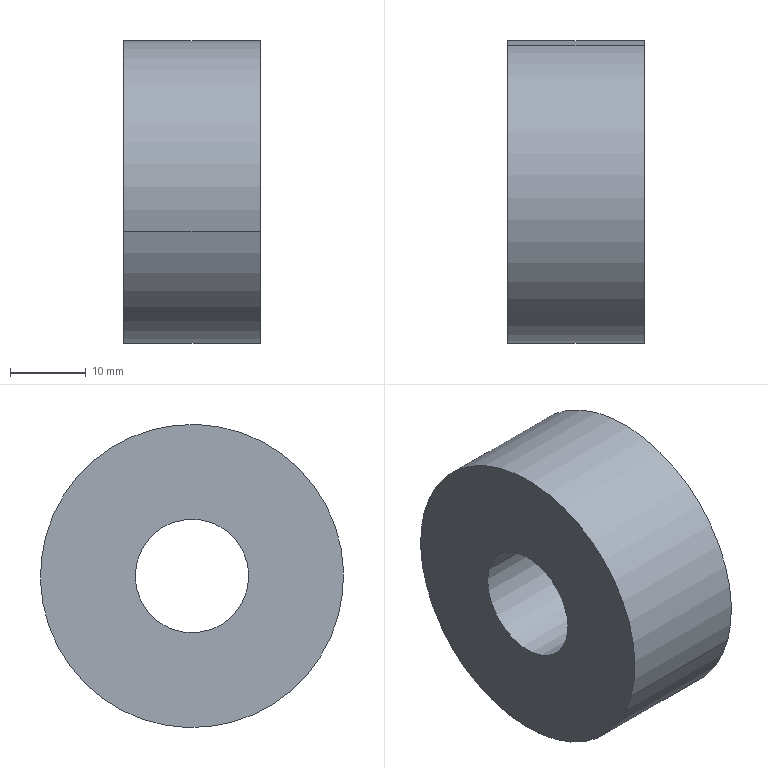Component | SolidWorks | NutRubberPad-1 | 1 solid | 6 faces | box 18 x 40 x 40 mm | volume 19439 mm3 | cylinder 4 | plane 2 | commonest cylinder face diameters 15 x2 40 x2
build123d program:
from build123d import *

# Parameters (mm, degrees)
SKETCH1_R           = 20
SKETCH1_R_2         = 7.5
BOSS_EXTRUDE1_DEPTH = 18


with BuildPart() as part:
    # Sketch1 → Boss-Extrude1 (new body)
    with BuildSketch(Plane.XY):
        Circle(SKETCH1_R)
        Circle(SKETCH1_R_2, mode=Mode.SUBTRACT)
    extrude(amount=BOSS_EXTRUDE1_DEPTH)


solid = part.part

# Placed as in the assembly
solid = solid.moved(Location((10.978, 19.945, 3.551), (0, 90, 0)))
STEP:
#1=CARTESIAN_POINT('',(1.141,0.5003,0.06227));
#2=VERTEX_POINT('',#1);
#3=CARTESIAN_POINT('',(1.141,1.07,0.2173));
#4=VERTEX_POINT('',#3);
#5=CARTESIAN_POINT('',(1.141,0.7853,0.1398));
#6=DIRECTION('',(1.,0.,-0.));
#7=DIRECTION('',(0.,0.9649,0.2625));
#8=AXIS2_PLACEMENT_3D('',#5,#6,#7);
#9=CIRCLE('',#8,0.2953);
#10=EDGE_CURVE('',#2,#4,#9,.T.);
#11=ORIENTED_EDGE('',*,*,#10,.T.);
#12=CARTESIAN_POINT('',(0.4322,1.07,0.2173));
#13=VERTEX_POINT('',#12);
#14=CARTESIAN_POINT('',(1.141,1.07,0.2173));
#15=DIRECTION('',(-1.,-0.,0.));
#16=VECTOR('',#15,39.37);
#17=LINE('',#14,#16);
#18=EDGE_CURVE('',#4,#13,#17,.T.);
#19=ORIENTED_EDGE('',*,*,#18,.T.);
#20=CARTESIAN_POINT('',(0.4322,0.5003,0.06227));
#21=VERTEX_POINT('',#20);
#22=CARTESIAN_POINT('',(0.4322,0.7853,0.1398));
#23=DIRECTION('',(1.,0.,-0.));
#24=DIRECTION('',(0.,0.9649,0.2625));
#25=AXIS2_PLACEMENT_3D('',#22,#23,#24);
#26=CIRCLE('',#25,0.2953);
#27=EDGE_CURVE('',#21,#13,#26,.T.);
#28=ORIENTED_EDGE('',*,*,#27,.F.);
#29=CARTESIAN_POINT('',(1.141,0.5003,0.06227));
#30=DIRECTION('',(-1.,-0.,0.));
#31=VECTOR('',#30,39.37);
#32=LINE('',#29,#31);
#33=EDGE_CURVE('',#2,#21,#32,.T.);
#34=ORIENTED_EDGE('',*,*,#33,.F.);
#35=EDGE_LOOP('',(#11,#19,#28,#34));
#36=FACE_OUTER_BOUND('',#35,.T.);
#37=CARTESIAN_POINT('',(1.141,0.7853,0.1398));
#38=DIRECTION('',(-1.,-0.,0.));
#39=DIRECTION('',(0.,-0.9649,-0.2625));
#40=AXIS2_PLACEMENT_3D('',#37,#38,#39);
#41=CYLINDRICAL_SURFACE('',#40,0.2953);
#42=ADVANCED_FACE('',(#36),#41,.F.);
#43=CARTESIAN_POINT('',(1.141,1.545,0.3465));
#44=VERTEX_POINT('',#43);
#45=CARTESIAN_POINT('',(1.141,0.02547,-0.06693));
#46=VERTEX_POINT('',#45);
#47=CARTESIAN_POINT('',(1.141,0.7853,0.1398));
#48=DIRECTION('',(1.,0.,-0.));
#49=DIRECTION('',(0.,0.9649,0.2625));
#50=AXIS2_PLACEMENT_3D('',#47,#48,#49);
#51=CIRCLE('',#50,0.7874);
#52=EDGE_CURVE('',#44,#46,#51,.T.);
#53=ORIENTED_EDGE('',*,*,#52,.F.);
#54=CARTESIAN_POINT('',(0.4322,1.545,0.3465));
#55=VERTEX_POINT('',#54);
#56=CARTESIAN_POINT('',(1.141,1.545,0.3465));
#57=DIRECTION('',(-1.,-0.,0.));
#58=VECTOR('',#57,39.37);
#59=LINE('',#56,#58);
#60=EDGE_CURVE('',#44,#55,#59,.T.);
#61=ORIENTED_EDGE('',*,*,#60,.T.);
#62=CARTESIAN_POINT('',(0.4322,0.02547,-0.06693));
#63=VERTEX_POINT('',#62);
#64=CARTESIAN_POINT('',(0.4322,0.7853,0.1398));
#65=DIRECTION('',(1.,0.,-0.));
#66=DIRECTION('',(0.,0.9649,0.2625));
#67=AXIS2_PLACEMENT_3D('',#64,#65,#66);
#68=CIRCLE('',#67,0.7874);
#69=EDGE_CURVE('',#55,#63,#68,.T.);
#70=ORIENTED_EDGE('',*,*,#69,.T.);
#71=CARTESIAN_POINT('',(1.141,0.02547,-0.06693));
#72=DIRECTION('',(-1.,-0.,0.));
#73=VECTOR('',#72,39.37);
#74=LINE('',#71,#73);
#75=EDGE_CURVE('',#46,#63,#74,.T.);
#76=ORIENTED_EDGE('',*,*,#75,.F.);
#77=EDGE_LOOP('',(#53,#61,#70,#76));
#78=FACE_OUTER_BOUND('',#77,.T.);
#79=CARTESIAN_POINT('',(1.141,0.7853,0.1398));
#80=DIRECTION('',(-1.,-0.,0.));
#81=DIRECTION('',(0.,-0.9649,-0.2625));
#82=AXIS2_PLACEMENT_3D('',#79,#80,#81);
#83=CYLINDRICAL_SURFACE('',#82,0.7874);
#84=ADVANCED_FACE('',(#78),#83,.T.);
#85=CARTESIAN_POINT('',(1.141,0.7853,0.1398));
#86=DIRECTION('',(1.,0.,-0.));
#87=DIRECTION('',(0.,0.9649,0.2625));
#88=AXIS2_PLACEMENT_3D('',#85,#86,#87);
#89=CIRCLE('',#88,0.7874);
#90=EDGE_CURVE('',#46,#44,#89,.T.);
#91=ORIENTED_EDGE('',*,*,#90,.T.);
#92=ORIENTED_EDGE('',*,*,#52,.T.);
#93=EDGE_LOOP('',(#91,#92));
#94=FACE_OUTER_BOUND('',#93,.T.);
#95=ORIENTED_EDGE('',*,*,#10,.F.);
#96=CARTESIAN_POINT('',(1.141,0.7853,0.1398));
#97=DIRECTION('',(1.,0.,-0.));
#98=DIRECTION('',(0.,0.9649,0.2625));
#99=AXIS2_PLACEMENT_3D('',#96,#97,#98);
#100=CIRCLE('',#99,0.2953);
#101=EDGE_CURVE('',#4,#2,#100,.T.);
#102=ORIENTED_EDGE('',*,*,#101,.F.);
#103=EDGE_LOOP('',(#95,#102));
#104=FACE_BOUND('',#103,.T.);
#105=CARTESIAN_POINT('',(1.141,0.7853,0.1398));
#106=DIRECTION('',(1.,0.,-0.));
#107=DIRECTION('',(0.,0.9649,0.2625));
#108=AXIS2_PLACEMENT_3D('',#105,#106,#107);
#109=PLANE('',#108);
#110=ADVANCED_FACE('',(#94,#104),#109,.T.);
#111=CARTESIAN_POINT('',(0.4322,0.7853,0.1398));
#112=DIRECTION('',(1.,0.,-0.));
#113=DIRECTION('',(0.,0.9649,0.2625));
#114=AXIS2_PLACEMENT_3D('',#111,#112,#113);
#115=CIRCLE('',#114,0.7874);
#116=EDGE_CURVE('',#63,#55,#115,.T.);
#117=ORIENTED_EDGE('',*,*,#116,.F.);
#118=ORIENTED_EDGE('',*,*,#69,.F.);
#119=EDGE_LOOP('',(#117,#118));
#120=FACE_OUTER_BOUND('',#119,.T.);
#121=ORIENTED_EDGE('',*,*,#27,.T.);
#122=CARTESIAN_POINT('',(0.4322,0.7853,0.1398));
#123=DIRECTION('',(1.,0.,-0.));
#124=DIRECTION('',(0.,0.9649,0.2625));
#125=AXIS2_PLACEMENT_3D('',#122,#123,#124);
#126=CIRCLE('',#125,0.2953);
#127=EDGE_CURVE('',#13,#21,#126,.T.);
#128=ORIENTED_EDGE('',*,*,#127,.T.);
#129=EDGE_LOOP('',(#121,#128));
#130=FACE_BOUND('',#129,.T.);
#131=CARTESIAN_POINT('',(0.4322,0.7853,0.1398));
#132=DIRECTION('',(1.,0.,-0.));
#133=DIRECTION('',(0.,0.9649,0.2625));
#134=AXIS2_PLACEMENT_3D('',#131,#132,#133);
#135=PLANE('',#134);
#136=ADVANCED_FACE('',(#120,#130),#135,.F.);
#137=ORIENTED_EDGE('',*,*,#60,.F.);
#138=ORIENTED_EDGE('',*,*,#90,.F.);
#139=ORIENTED_EDGE('',*,*,#75,.T.);
#140=ORIENTED_EDGE('',*,*,#116,.T.);
#141=EDGE_LOOP('',(#137,#138,#139,#140));
#142=FACE_OUTER_BOUND('',#141,.T.);
#143=CARTESIAN_POINT('',(1.141,0.7853,0.1398));
#144=DIRECTION('',(-1.,-0.,0.));
#145=DIRECTION('',(0.,-0.9649,-0.2625));
#146=AXIS2_PLACEMENT_3D('',#143,#144,#145);
#147=CYLINDRICAL_SURFACE('',#146,0.7874);
#148=ADVANCED_FACE('',(#142),#147,.T.);
#149=ORIENTED_EDGE('',*,*,#18,.F.);
#150=ORIENTED_EDGE('',*,*,#101,.T.);
#151=ORIENTED_EDGE('',*,*,#33,.T.);
#152=ORIENTED_EDGE('',*,*,#127,.F.);
#153=EDGE_LOOP('',(#149,#150,#151,#152));
#154=FACE_OUTER_BOUND('',#153,.T.);
#155=CARTESIAN_POINT('',(1.141,0.7853,0.1398));
#156=DIRECTION('',(-1.,-0.,0.));
#157=DIRECTION('',(0.,-0.9649,-0.2625));
#158=AXIS2_PLACEMENT_3D('',#155,#156,#157);
#159=CYLINDRICAL_SURFACE('',#158,0.2953);
#160=ADVANCED_FACE('',(#154),#159,.F.);
#161=CLOSED_SHELL('',(#42,#84,#110,#136,#148,#160));
#162=MANIFOLD_SOLID_BREP('',#161);
#163=CARTESIAN_POINT('',(0.,0.,0.));
#164=DIRECTION('',(0.,0.,1.));
#165=DIRECTION('',(1.,0.,0.));
#166=AXIS2_PLACEMENT_3D('',#163,#164,#165);
#167=(LENGTH_UNIT()NAMED_UNIT(*)SI_UNIT($,.METRE.));
#168=LENGTH_MEASURE_WITH_UNIT(LENGTH_MEASURE(0.0254),#167);
#169=DIMENSIONAL_EXPONENTS(1.,0.,0.,0.,0.,0.,0.);
#170=(CONVERSION_BASED_UNIT('',#168)LENGTH_UNIT()NAMED_UNIT(#169));
#171=UNCERTAINTY_MEASURE_WITH_UNIT(LENGTH_MEASURE(0.00001),#170,'','');
#172=(NAMED_UNIT(*)PLANE_ANGLE_UNIT()SI_UNIT($,.RADIAN.));
#173=(NAMED_UNIT(*)SI_UNIT($,.STERADIAN.)SOLID_ANGLE_UNIT());
#174=(GEOMETRIC_REPRESENTATION_CONTEXT(3)GLOBAL_UNCERTAINTY_ASSIGNED_CONTEXT((#171))GLOBAL_UNIT_ASSIGNED_CONTEXT((#170,#172,#173))REPRESENTATION_CONTEXT('',''));
#175=ADVANCED_BREP_SHAPE_REPRESENTATION('',(#162,#166),#174);
#176=COLOUR_RGB('',0.7922,0.8196,0.9333);
#177=FILL_AREA_STYLE_COLOUR('',#176);
#178=FILL_AREA_STYLE('',(#177));
#179=SURFACE_STYLE_FILL_AREA(#178);
#180=SURFACE_SIDE_STYLE('',(#179));
#181=SURFACE_STYLE_USAGE(.BOTH.,#180);
#182=PRESENTATION_STYLE_ASSIGNMENT((#181));
#183=STYLED_ITEM('',(#182),#162);
#184=(LENGTH_UNIT()NAMED_UNIT(*)SI_UNIT($,.METRE.));
#185=LENGTH_MEASURE_WITH_UNIT(LENGTH_MEASURE(0.0254),#184);
#186=DIMENSIONAL_EXPONENTS(1.,0.,0.,0.,0.,0.,0.);
#187=(CONVERSION_BASED_UNIT('',#185)LENGTH_UNIT()NAMED_UNIT(#186));
#188=UNCERTAINTY_MEASURE_WITH_UNIT(LENGTH_MEASURE(0.00001),#187,'','');
#189=(NAMED_UNIT(*)PLANE_ANGLE_UNIT()SI_UNIT($,.RADIAN.));
#190=(NAMED_UNIT(*)SI_UNIT($,.STERADIAN.)SOLID_ANGLE_UNIT());
#191=(GEOMETRIC_REPRESENTATION_CONTEXT(3)GLOBAL_UNCERTAINTY_ASSIGNED_CONTEXT((#188))GLOBAL_UNIT_ASSIGNED_CONTEXT((#187,#189,#190))REPRESENTATION_CONTEXT('',''));
#192=MECHANICAL_DESIGN_GEOMETRIC_PRESENTATION_REPRESENTATION('',(#183),#191);
#193=PRESENTATION_LAYER_ASSIGNMENT('','',(#183));